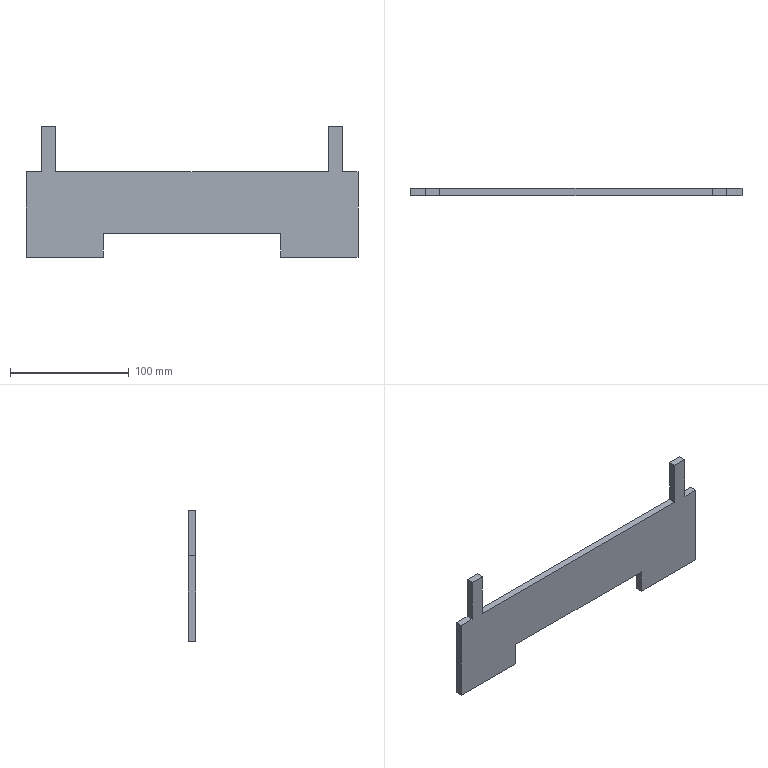Component | SolidWorks | THK-B1012LowerBaffle-1 | 1 solid | 18 faces | box 280 x 6 x 110 mm | volume 108432 mm3 | plane 18 | material Q235A
STEP:
#1=COLOUR_RGB('',0.7922,0.8196,0.9333);
#2=FILL_AREA_STYLE_COLOUR('',#1);
#3=FILL_AREA_STYLE('',(#2));
#4=SURFACE_STYLE_FILL_AREA(#3);
#5=SURFACE_SIDE_STYLE('',(#4));
#6=SURFACE_STYLE_USAGE(.BOTH.,#5);
#7=PRESENTATION_STYLE_ASSIGNMENT((#6));
#8=CARTESIAN_POINT('',(-5.,-5.354,-5.709));
#9=VERTEX_POINT('',#8);
#10=CARTESIAN_POINT('',(-4.528,-5.354,-5.709));
#11=VERTEX_POINT('',#10);
#12=CARTESIAN_POINT('',(-5.512,-5.354,-5.709));
#13=DIRECTION('',(1.,0.,0.));
#14=VECTOR('',#13,39.37);
#15=LINE('',#12,#14);
#16=EDGE_CURVE('',#9,#11,#15,.T.);
#17=ORIENTED_EDGE('',*,*,#16,.T.);
#18=CARTESIAN_POINT('',(-4.528,-5.118,-5.709));
#19=VERTEX_POINT('',#18);
#20=CARTESIAN_POINT('',(-4.528,-5.118,-5.709));
#21=DIRECTION('',(-0.,1.,0.));
#22=VECTOR('',#21,39.37);
#23=LINE('',#20,#22);
#24=EDGE_CURVE('',#11,#19,#23,.T.);
#25=ORIENTED_EDGE('',*,*,#24,.T.);
#26=CARTESIAN_POINT('',(-5.,-5.118,-5.709));
#27=VERTEX_POINT('',#26);
#28=CARTESIAN_POINT('',(-5.512,-5.118,-5.709));
#29=DIRECTION('',(1.,0.,0.));
#30=VECTOR('',#29,39.37);
#31=LINE('',#28,#30);
#32=EDGE_CURVE('',#27,#19,#31,.T.);
#33=ORIENTED_EDGE('',*,*,#32,.F.);
#34=CARTESIAN_POINT('',(-5.,-5.354,-5.709));
#35=DIRECTION('',(-0.,1.,0.));
#36=VECTOR('',#35,39.37);
#37=LINE('',#34,#36);
#38=EDGE_CURVE('',#9,#27,#37,.T.);
#39=ORIENTED_EDGE('',*,*,#38,.F.);
#40=EDGE_LOOP('',(#17,#25,#33,#39));
#41=FACE_OUTER_BOUND('',#40,.T.);
#42=CARTESIAN_POINT('',(0.,-5.118,-5.709));
#43=DIRECTION('',(0.,0.,-1.));
#44=DIRECTION('',(-1.,0.,0.));
#45=AXIS2_PLACEMENT_3D('',#42,#43,#44);
#46=PLANE('',#45);
#47=ADVANCED_FACE('',(#41),#46,.F.);
#48=CARTESIAN_POINT('',(-2.953,-5.354,-10.039));
#49=VERTEX_POINT('',#48);
#50=CARTESIAN_POINT('',(-2.953,-5.118,-10.039));
#51=VERTEX_POINT('',#50);
#52=CARTESIAN_POINT('',(-2.953,-5.118,-10.039));
#53=DIRECTION('',(-0.,1.,0.));
#54=VECTOR('',#53,39.37);
#55=LINE('',#52,#54);
#56=EDGE_CURVE('',#49,#51,#55,.T.);
#57=ORIENTED_EDGE('',*,*,#56,.F.);
#58=CARTESIAN_POINT('',(-5.512,-5.354,-10.039));
#59=VERTEX_POINT('',#58);
#60=CARTESIAN_POINT('',(-5.512,-5.354,-10.039));
#61=DIRECTION('',(1.,0.,0.));
#62=VECTOR('',#61,39.37);
#63=LINE('',#60,#62);
#64=EDGE_CURVE('',#59,#49,#63,.T.);
#65=ORIENTED_EDGE('',*,*,#64,.F.);
#66=CARTESIAN_POINT('',(-5.512,-5.118,-10.039));
#67=VERTEX_POINT('',#66);
#68=CARTESIAN_POINT('',(-5.512,-5.354,-10.039));
#69=DIRECTION('',(0.,1.,0.));
#70=VECTOR('',#69,39.37);
#71=LINE('',#68,#70);
#72=EDGE_CURVE('',#59,#67,#71,.T.);
#73=ORIENTED_EDGE('',*,*,#72,.T.);
#74=CARTESIAN_POINT('',(-5.512,-5.118,-10.039));
#75=DIRECTION('',(1.,0.,0.));
#76=VECTOR('',#75,39.37);
#77=LINE('',#74,#76);
#78=EDGE_CURVE('',#67,#51,#77,.T.);
#79=ORIENTED_EDGE('',*,*,#78,.T.);
#80=EDGE_LOOP('',(#57,#65,#73,#79));
#81=FACE_OUTER_BOUND('',#80,.T.);
#82=CARTESIAN_POINT('',(0.,-5.118,-10.039));
#83=DIRECTION('',(0.,0.,-1.));
#84=DIRECTION('',(-1.,0.,0.));
#85=AXIS2_PLACEMENT_3D('',#82,#83,#84);
#86=PLANE('',#85);
#87=ADVANCED_FACE('',(#81),#86,.T.);
#88=CARTESIAN_POINT('',(5.512,-5.354,-7.205));
#89=VERTEX_POINT('',#88);
#90=CARTESIAN_POINT('',(5.,-5.354,-7.205));
#91=VERTEX_POINT('',#90);
#92=CARTESIAN_POINT('',(5.512,-5.354,-7.205));
#93=DIRECTION('',(-1.,-0.,0.));
#94=VECTOR('',#93,39.37);
#95=LINE('',#92,#94);
#96=EDGE_CURVE('',#89,#91,#95,.T.);
#97=ORIENTED_EDGE('',*,*,#96,.T.);
#98=CARTESIAN_POINT('',(5.,-5.354,-5.709));
#99=VERTEX_POINT('',#98);
#100=CARTESIAN_POINT('',(5.,-5.354,-5.709));
#101=DIRECTION('',(0.,0.,1.));
#102=VECTOR('',#101,39.37);
#103=LINE('',#100,#102);
#104=EDGE_CURVE('',#91,#99,#103,.T.);
#105=ORIENTED_EDGE('',*,*,#104,.T.);
#106=CARTESIAN_POINT('',(4.528,-5.354,-5.709));
#107=VERTEX_POINT('',#106);
#108=CARTESIAN_POINT('',(-5.512,-5.354,-5.709));
#109=DIRECTION('',(1.,0.,0.));
#110=VECTOR('',#109,39.37);
#111=LINE('',#108,#110);
#112=EDGE_CURVE('',#107,#99,#111,.T.);
#113=ORIENTED_EDGE('',*,*,#112,.F.);
#114=CARTESIAN_POINT('',(4.528,-5.354,-7.205));
#115=VERTEX_POINT('',#114);
#116=CARTESIAN_POINT('',(4.528,-5.354,-7.205));
#117=DIRECTION('',(0.,0.,-1.));
#118=VECTOR('',#117,39.37);
#119=LINE('',#116,#118);
#120=EDGE_CURVE('',#107,#115,#119,.T.);
#121=ORIENTED_EDGE('',*,*,#120,.T.);
#122=CARTESIAN_POINT('',(-4.528,-5.354,-7.205));
#123=VERTEX_POINT('',#122);
#124=CARTESIAN_POINT('',(-4.528,-5.354,-7.205));
#125=DIRECTION('',(-1.,-0.,0.));
#126=VECTOR('',#125,39.37);
#127=LINE('',#124,#126);
#128=EDGE_CURVE('',#115,#123,#127,.T.);
#129=ORIENTED_EDGE('',*,*,#128,.T.);
#130=CARTESIAN_POINT('',(-4.528,-5.354,-7.205));
#131=DIRECTION('',(0.,0.,1.));
#132=VECTOR('',#131,39.37);
#133=LINE('',#130,#132);
#134=EDGE_CURVE('',#123,#11,#133,.T.);
#135=ORIENTED_EDGE('',*,*,#134,.T.);
#136=ORIENTED_EDGE('',*,*,#16,.F.);
#137=CARTESIAN_POINT('',(-5.,-5.354,-7.205));
#138=VERTEX_POINT('',#137);
#139=CARTESIAN_POINT('',(-5.,-5.354,-5.709));
#140=DIRECTION('',(0.,0.,-1.));
#141=VECTOR('',#140,39.37);
#142=LINE('',#139,#141);
#143=EDGE_CURVE('',#9,#138,#142,.T.);
#144=ORIENTED_EDGE('',*,*,#143,.T.);
#145=CARTESIAN_POINT('',(-5.512,-5.354,-7.205));
#146=VERTEX_POINT('',#145);
#147=CARTESIAN_POINT('',(-5.512,-5.354,-7.205));
#148=DIRECTION('',(-1.,-0.,0.));
#149=VECTOR('',#148,39.37);
#150=LINE('',#147,#149);
#151=EDGE_CURVE('',#138,#146,#150,.T.);
#152=ORIENTED_EDGE('',*,*,#151,.T.);
#153=CARTESIAN_POINT('',(-5.512,-5.354,-5.709));
#154=DIRECTION('',(0.,0.,-1.));
#155=VECTOR('',#154,39.37);
#156=LINE('',#153,#155);
#157=EDGE_CURVE('',#146,#59,#156,.T.);
#158=ORIENTED_EDGE('',*,*,#157,.T.);
#159=ORIENTED_EDGE('',*,*,#64,.T.);
#160=CARTESIAN_POINT('',(-2.953,-5.354,-9.252));
#161=VERTEX_POINT('',#160);
#162=CARTESIAN_POINT('',(-2.953,-5.354,-9.252));
#163=DIRECTION('',(0.,0.,1.));
#164=VECTOR('',#163,39.37);
#165=LINE('',#162,#164);
#166=EDGE_CURVE('',#49,#161,#165,.T.);
#167=ORIENTED_EDGE('',*,*,#166,.T.);
#168=CARTESIAN_POINT('',(2.953,-5.354,-9.252));
#169=VERTEX_POINT('',#168);
#170=CARTESIAN_POINT('',(-2.953,-5.354,-9.252));
#171=DIRECTION('',(1.,0.,0.));
#172=VECTOR('',#171,39.37);
#173=LINE('',#170,#172);
#174=EDGE_CURVE('',#161,#169,#173,.T.);
#175=ORIENTED_EDGE('',*,*,#174,.T.);
#176=CARTESIAN_POINT('',(2.953,-5.354,-10.039));
#177=VERTEX_POINT('',#176);
#178=CARTESIAN_POINT('',(2.953,-5.354,-9.252));
#179=DIRECTION('',(0.,0.,-1.));
#180=VECTOR('',#179,39.37);
#181=LINE('',#178,#180);
#182=EDGE_CURVE('',#169,#177,#181,.T.);
#183=ORIENTED_EDGE('',*,*,#182,.T.);
#184=CARTESIAN_POINT('',(5.512,-5.354,-10.039));
#185=VERTEX_POINT('',#184);
#186=CARTESIAN_POINT('',(-5.512,-5.354,-10.039));
#187=DIRECTION('',(1.,0.,0.));
#188=VECTOR('',#187,39.37);
#189=LINE('',#186,#188);
#190=EDGE_CURVE('',#177,#185,#189,.T.);
#191=ORIENTED_EDGE('',*,*,#190,.T.);
#192=CARTESIAN_POINT('',(5.512,-5.354,-5.709));
#193=DIRECTION('',(0.,0.,-1.));
#194=VECTOR('',#193,39.37);
#195=LINE('',#192,#194);
#196=EDGE_CURVE('',#89,#185,#195,.T.);
#197=ORIENTED_EDGE('',*,*,#196,.F.);
#198=EDGE_LOOP('',(#97,#105,#113,#121,#129,#135,#136,#144,#152,#158,#159,#167,#175,#183,#191,#197));
#199=FACE_OUTER_BOUND('',#198,.T.);
#200=CARTESIAN_POINT('',(-5.512,-5.354,-5.709));
#201=DIRECTION('',(-0.,1.,0.));
#202=DIRECTION('',(-1.,-0.,0.));
#203=AXIS2_PLACEMENT_3D('',#200,#201,#202);
#204=PLANE('',#203);
#205=ADVANCED_FACE('',(#199),#204,.F.);
#206=CARTESIAN_POINT('',(5.512,-5.118,-7.205));
#207=VERTEX_POINT('',#206);
#208=CARTESIAN_POINT('',(5.512,-5.354,-7.205));
#209=DIRECTION('',(-0.,1.,0.));
#210=VECTOR('',#209,39.37);
#211=LINE('',#208,#210);
#212=EDGE_CURVE('',#89,#207,#211,.T.);
#213=ORIENTED_EDGE('',*,*,#212,.F.);
#214=ORIENTED_EDGE('',*,*,#196,.T.);
#215=CARTESIAN_POINT('',(5.512,-5.118,-10.039));
#216=VERTEX_POINT('',#215);
#217=CARTESIAN_POINT('',(5.512,-5.118,-10.039));
#218=DIRECTION('',(0.,-1.,0.));
#219=VECTOR('',#218,39.37);
#220=LINE('',#217,#219);
#221=EDGE_CURVE('',#216,#185,#220,.T.);
#222=ORIENTED_EDGE('',*,*,#221,.F.);
#223=CARTESIAN_POINT('',(5.512,-5.118,-5.709));
#224=DIRECTION('',(0.,0.,-1.));
#225=VECTOR('',#224,39.37);
#226=LINE('',#223,#225);
#227=EDGE_CURVE('',#207,#216,#226,.T.);
#228=ORIENTED_EDGE('',*,*,#227,.F.);
#229=EDGE_LOOP('',(#213,#214,#222,#228));
#230=FACE_OUTER_BOUND('',#229,.T.);
#231=CARTESIAN_POINT('',(5.512,-5.118,-5.709));
#232=DIRECTION('',(1.,0.,0.));
#233=DIRECTION('',(0.,0.,-1.));
#234=AXIS2_PLACEMENT_3D('',#231,#232,#233);
#235=PLANE('',#234);
#236=ADVANCED_FACE('',(#230),#235,.T.);
#237=CARTESIAN_POINT('',(5.,-5.118,-7.205));
#238=VERTEX_POINT('',#237);
#239=CARTESIAN_POINT('',(5.,-5.118,-5.709));
#240=VERTEX_POINT('',#239);
#241=CARTESIAN_POINT('',(5.,-5.118,-5.709));
#242=DIRECTION('',(0.,0.,1.));
#243=VECTOR('',#242,39.37);
#244=LINE('',#241,#243);
#245=EDGE_CURVE('',#238,#240,#244,.T.);
#246=ORIENTED_EDGE('',*,*,#245,.F.);
#247=CARTESIAN_POINT('',(5.512,-5.118,-7.205));
#248=DIRECTION('',(-1.,-0.,0.));
#249=VECTOR('',#248,39.37);
#250=LINE('',#247,#249);
#251=EDGE_CURVE('',#207,#238,#250,.T.);
#252=ORIENTED_EDGE('',*,*,#251,.F.);
#253=ORIENTED_EDGE('',*,*,#227,.T.);
#254=CARTESIAN_POINT('',(2.953,-5.118,-10.039));
#255=VERTEX_POINT('',#254);
#256=CARTESIAN_POINT('',(-5.512,-5.118,-10.039));
#257=DIRECTION('',(1.,0.,0.));
#258=VECTOR('',#257,39.37);
#259=LINE('',#256,#258);
#260=EDGE_CURVE('',#255,#216,#259,.T.);
#261=ORIENTED_EDGE('',*,*,#260,.F.);
#262=CARTESIAN_POINT('',(2.953,-5.118,-9.252));
#263=VERTEX_POINT('',#262);
#264=CARTESIAN_POINT('',(2.953,-5.118,-9.252));
#265=DIRECTION('',(0.,0.,-1.));
#266=VECTOR('',#265,39.37);
#267=LINE('',#264,#266);
#268=EDGE_CURVE('',#263,#255,#267,.T.);
#269=ORIENTED_EDGE('',*,*,#268,.F.);
#270=CARTESIAN_POINT('',(-2.953,-5.118,-9.252));
#271=VERTEX_POINT('',#270);
#272=CARTESIAN_POINT('',(-2.953,-5.118,-9.252));
#273=DIRECTION('',(1.,0.,0.));
#274=VECTOR('',#273,39.37);
#275=LINE('',#272,#274);
#276=EDGE_CURVE('',#271,#263,#275,.T.);
#277=ORIENTED_EDGE('',*,*,#276,.F.);
#278=CARTESIAN_POINT('',(-2.953,-5.118,-9.252));
#279=DIRECTION('',(0.,0.,1.));
#280=VECTOR('',#279,39.37);
#281=LINE('',#278,#280);
#282=EDGE_CURVE('',#51,#271,#281,.T.);
#283=ORIENTED_EDGE('',*,*,#282,.F.);
#284=ORIENTED_EDGE('',*,*,#78,.F.);
#285=CARTESIAN_POINT('',(-5.512,-5.118,-7.205));
#286=VERTEX_POINT('',#285);
#287=CARTESIAN_POINT('',(-5.512,-5.118,-5.709));
#288=DIRECTION('',(0.,0.,-1.));
#289=VECTOR('',#288,39.37);
#290=LINE('',#287,#289);
#291=EDGE_CURVE('',#286,#67,#290,.T.);
#292=ORIENTED_EDGE('',*,*,#291,.F.);
#293=CARTESIAN_POINT('',(-5.,-5.118,-7.205));
#294=VERTEX_POINT('',#293);
#295=CARTESIAN_POINT('',(-5.512,-5.118,-7.205));
#296=DIRECTION('',(-1.,-0.,0.));
#297=VECTOR('',#296,39.37);
#298=LINE('',#295,#297);
#299=EDGE_CURVE('',#294,#286,#298,.T.);
#300=ORIENTED_EDGE('',*,*,#299,.F.);
#301=CARTESIAN_POINT('',(-5.,-5.118,-5.709));
#302=DIRECTION('',(0.,0.,-1.));
#303=VECTOR('',#302,39.37);
#304=LINE('',#301,#303);
#305=EDGE_CURVE('',#27,#294,#304,.T.);
#306=ORIENTED_EDGE('',*,*,#305,.F.);
#307=ORIENTED_EDGE('',*,*,#32,.T.);
#308=CARTESIAN_POINT('',(-4.528,-5.118,-7.205));
#309=VERTEX_POINT('',#308);
#310=CARTESIAN_POINT('',(-4.528,-5.118,-7.205));
#311=DIRECTION('',(0.,0.,1.));
#312=VECTOR('',#311,39.37);
#313=LINE('',#310,#312);
#314=EDGE_CURVE('',#309,#19,#313,.T.);
#315=ORIENTED_EDGE('',*,*,#314,.F.);
#316=CARTESIAN_POINT('',(4.528,-5.118,-7.205));
#317=VERTEX_POINT('',#316);
#318=CARTESIAN_POINT('',(-4.528,-5.118,-7.205));
#319=DIRECTION('',(-1.,-0.,0.));
#320=VECTOR('',#319,39.37);
#321=LINE('',#318,#320);
#322=EDGE_CURVE('',#317,#309,#321,.T.);
#323=ORIENTED_EDGE('',*,*,#322,.F.);
#324=CARTESIAN_POINT('',(4.528,-5.118,-5.709));
#325=VERTEX_POINT('',#324);
#326=CARTESIAN_POINT('',(4.528,-5.118,-7.205));
#327=DIRECTION('',(0.,0.,-1.));
#328=VECTOR('',#327,39.37);
#329=LINE('',#326,#328);
#330=EDGE_CURVE('',#325,#317,#329,.T.);
#331=ORIENTED_EDGE('',*,*,#330,.F.);
#332=CARTESIAN_POINT('',(-5.512,-5.118,-5.709));
#333=DIRECTION('',(1.,0.,0.));
#334=VECTOR('',#333,39.37);
#335=LINE('',#332,#334);
#336=EDGE_CURVE('',#325,#240,#335,.T.);
#337=ORIENTED_EDGE('',*,*,#336,.T.);
#338=EDGE_LOOP('',(#246,#252,#253,#261,#269,#277,#283,#284,#292,#300,#306,#307,#315,#323,#331,#337));
#339=FACE_OUTER_BOUND('',#338,.T.);
#340=CARTESIAN_POINT('',(-5.512,-5.118,-5.709));
#341=DIRECTION('',(-0.,1.,0.));
#342=DIRECTION('',(-1.,-0.,0.));
#343=AXIS2_PLACEMENT_3D('',#340,#341,#342);
#344=PLANE('',#343);
#345=ADVANCED_FACE('',(#339),#344,.T.);
#346=CARTESIAN_POINT('',(-5.512,-5.354,-7.205));
#347=DIRECTION('',(-0.,1.,0.));
#348=VECTOR('',#347,39.37);
#349=LINE('',#346,#348);
#350=EDGE_CURVE('',#146,#286,#349,.T.);
#351=ORIENTED_EDGE('',*,*,#350,.T.);
#352=ORIENTED_EDGE('',*,*,#291,.T.);
#353=ORIENTED_EDGE('',*,*,#72,.F.);
#354=ORIENTED_EDGE('',*,*,#157,.F.);
#355=EDGE_LOOP('',(#351,#352,#353,#354));
#356=FACE_OUTER_BOUND('',#355,.T.);
#357=CARTESIAN_POINT('',(-5.512,-5.354,-5.709));
#358=DIRECTION('',(-1.,0.,0.));
#359=DIRECTION('',(0.,0.,1.));
#360=AXIS2_PLACEMENT_3D('',#357,#358,#359);
#361=PLANE('',#360);
#362=ADVANCED_FACE('',(#356),#361,.T.);
#363=ORIENTED_EDGE('',*,*,#112,.T.);
#364=CARTESIAN_POINT('',(5.,-5.354,-5.709));
#365=DIRECTION('',(-0.,1.,0.));
#366=VECTOR('',#365,39.37);
#367=LINE('',#364,#366);
#368=EDGE_CURVE('',#99,#240,#367,.T.);
#369=ORIENTED_EDGE('',*,*,#368,.T.);
#370=ORIENTED_EDGE('',*,*,#336,.F.);
#371=CARTESIAN_POINT('',(4.528,-5.118,-5.709));
#372=DIRECTION('',(0.,-1.,0.));
#373=VECTOR('',#372,39.37);
#374=LINE('',#371,#373);
#375=EDGE_CURVE('',#325,#107,#374,.T.);
#376=ORIENTED_EDGE('',*,*,#375,.T.);
#377=EDGE_LOOP('',(#363,#369,#370,#376));
#378=FACE_OUTER_BOUND('',#377,.T.);
#379=CARTESIAN_POINT('',(0.,-5.118,-5.709));
#380=DIRECTION('',(0.,0.,-1.));
#381=DIRECTION('',(-1.,0.,0.));
#382=AXIS2_PLACEMENT_3D('',#379,#380,#381);
#383=PLANE('',#382);
#384=ADVANCED_FACE('',(#378),#383,.F.);
#385=CARTESIAN_POINT('',(2.953,-5.118,-10.039));
#386=DIRECTION('',(0.,-1.,0.));
#387=VECTOR('',#386,39.37);
#388=LINE('',#385,#387);
#389=EDGE_CURVE('',#255,#177,#388,.T.);
#390=ORIENTED_EDGE('',*,*,#389,.F.);
#391=ORIENTED_EDGE('',*,*,#260,.T.);
#392=ORIENTED_EDGE('',*,*,#221,.T.);
#393=ORIENTED_EDGE('',*,*,#190,.F.);
#394=EDGE_LOOP('',(#390,#391,#392,#393));
#395=FACE_OUTER_BOUND('',#394,.T.);
#396=CARTESIAN_POINT('',(0.,-5.118,-10.039));
#397=DIRECTION('',(0.,0.,-1.));
#398=DIRECTION('',(-1.,0.,0.));
#399=AXIS2_PLACEMENT_3D('',#396,#397,#398);
#400=PLANE('',#399);
#401=ADVANCED_FACE('',(#395),#400,.T.);
#402=ORIENTED_EDGE('',*,*,#56,.T.);
#403=ORIENTED_EDGE('',*,*,#282,.T.);
#404=CARTESIAN_POINT('',(-2.953,-5.354,-9.252));
#405=DIRECTION('',(-0.,1.,0.));
#406=VECTOR('',#405,39.37);
#407=LINE('',#404,#406);
#408=EDGE_CURVE('',#161,#271,#407,.T.);
#409=ORIENTED_EDGE('',*,*,#408,.F.);
#410=ORIENTED_EDGE('',*,*,#166,.F.);
#411=EDGE_LOOP('',(#402,#403,#409,#410));
#412=FACE_OUTER_BOUND('',#411,.T.);
#413=CARTESIAN_POINT('',(-2.953,-5.354,-9.252));
#414=DIRECTION('',(-1.,-0.,0.));
#415=DIRECTION('',(0.,-1.,0.));
#416=AXIS2_PLACEMENT_3D('',#413,#414,#415);
#417=PLANE('',#416);
#418=ADVANCED_FACE('',(#412),#417,.F.);
#419=ORIENTED_EDGE('',*,*,#389,.T.);
#420=ORIENTED_EDGE('',*,*,#182,.F.);
#421=CARTESIAN_POINT('',(2.953,-5.354,-9.252));
#422=DIRECTION('',(-0.,1.,0.));
#423=VECTOR('',#422,39.37);
#424=LINE('',#421,#423);
#425=EDGE_CURVE('',#169,#263,#424,.T.);
#426=ORIENTED_EDGE('',*,*,#425,.T.);
#427=ORIENTED_EDGE('',*,*,#268,.T.);
#428=EDGE_LOOP('',(#419,#420,#426,#427));
#429=FACE_OUTER_BOUND('',#428,.T.);
#430=CARTESIAN_POINT('',(2.953,-5.354,-9.252));
#431=DIRECTION('',(1.,0.,0.));
#432=DIRECTION('',(-0.,1.,0.));
#433=AXIS2_PLACEMENT_3D('',#430,#431,#432);
#434=PLANE('',#433);
#435=ADVANCED_FACE('',(#429),#434,.F.);
#436=ORIENTED_EDGE('',*,*,#276,.T.);
#437=ORIENTED_EDGE('',*,*,#425,.F.);
#438=ORIENTED_EDGE('',*,*,#174,.F.);
#439=ORIENTED_EDGE('',*,*,#408,.T.);
#440=EDGE_LOOP('',(#436,#437,#438,#439));
#441=FACE_OUTER_BOUND('',#440,.T.);
#442=CARTESIAN_POINT('',(-2.953,-5.354,-9.252));
#443=DIRECTION('',(0.,0.,1.));
#444=DIRECTION('',(1.,0.,0.));
#445=AXIS2_PLACEMENT_3D('',#442,#443,#444);
#446=PLANE('',#445);
#447=ADVANCED_FACE('',(#441),#446,.F.);
#448=ORIENTED_EDGE('',*,*,#299,.T.);
#449=ORIENTED_EDGE('',*,*,#350,.F.);
#450=ORIENTED_EDGE('',*,*,#151,.F.);
#451=CARTESIAN_POINT('',(-5.,-5.354,-7.205));
#452=DIRECTION('',(-0.,1.,0.));
#453=VECTOR('',#452,39.37);
#454=LINE('',#451,#453);
#455=EDGE_CURVE('',#138,#294,#454,.T.);
#456=ORIENTED_EDGE('',*,*,#455,.T.);
#457=EDGE_LOOP('',(#448,#449,#450,#456));
#458=FACE_OUTER_BOUND('',#457,.T.);
#459=CARTESIAN_POINT('',(-5.512,-5.354,-7.205));
#460=DIRECTION('',(0.,0.,-1.));
#461=DIRECTION('',(-1.,0.,0.));
#462=AXIS2_PLACEMENT_3D('',#459,#460,#461);
#463=PLANE('',#462);
#464=ADVANCED_FACE('',(#458),#463,.F.);
#465=ORIENTED_EDGE('',*,*,#305,.T.);
#466=ORIENTED_EDGE('',*,*,#455,.F.);
#467=ORIENTED_EDGE('',*,*,#143,.F.);
#468=ORIENTED_EDGE('',*,*,#38,.T.);
#469=EDGE_LOOP('',(#465,#466,#467,#468));
#470=FACE_OUTER_BOUND('',#469,.T.);
#471=CARTESIAN_POINT('',(-5.,-5.354,-5.709));
#472=DIRECTION('',(1.,0.,0.));
#473=DIRECTION('',(-0.,1.,0.));
#474=AXIS2_PLACEMENT_3D('',#471,#472,#473);
#475=PLANE('',#474);
#476=ADVANCED_FACE('',(#470),#475,.F.);
#477=ORIENTED_EDGE('',*,*,#134,.F.);
#478=CARTESIAN_POINT('',(-4.528,-5.354,-7.205));
#479=DIRECTION('',(-0.,1.,0.));
#480=VECTOR('',#479,39.37);
#481=LINE('',#478,#480);
#482=EDGE_CURVE('',#123,#309,#481,.T.);
#483=ORIENTED_EDGE('',*,*,#482,.T.);
#484=ORIENTED_EDGE('',*,*,#314,.T.);
#485=ORIENTED_EDGE('',*,*,#24,.F.);
#486=EDGE_LOOP('',(#477,#483,#484,#485));
#487=FACE_OUTER_BOUND('',#486,.T.);
#488=CARTESIAN_POINT('',(-4.528,-5.354,-7.205));
#489=DIRECTION('',(-1.,-0.,0.));
#490=DIRECTION('',(0.,0.,1.));
#491=AXIS2_PLACEMENT_3D('',#488,#489,#490);
#492=PLANE('',#491);
#493=ADVANCED_FACE('',(#487),#492,.F.);
#494=ORIENTED_EDGE('',*,*,#330,.T.);
#495=CARTESIAN_POINT('',(4.528,-5.354,-7.205));
#496=DIRECTION('',(-0.,1.,0.));
#497=VECTOR('',#496,39.37);
#498=LINE('',#495,#497);
#499=EDGE_CURVE('',#115,#317,#498,.T.);
#500=ORIENTED_EDGE('',*,*,#499,.F.);
#501=ORIENTED_EDGE('',*,*,#120,.F.);
#502=ORIENTED_EDGE('',*,*,#375,.F.);
#503=EDGE_LOOP('',(#494,#500,#501,#502));
#504=FACE_OUTER_BOUND('',#503,.T.);
#505=CARTESIAN_POINT('',(4.528,-5.354,-7.205));
#506=DIRECTION('',(1.,0.,0.));
#507=DIRECTION('',(0.,0.,-1.));
#508=AXIS2_PLACEMENT_3D('',#505,#506,#507);
#509=PLANE('',#508);
#510=ADVANCED_FACE('',(#504),#509,.F.);
#511=ORIENTED_EDGE('',*,*,#322,.T.);
#512=ORIENTED_EDGE('',*,*,#482,.F.);
#513=ORIENTED_EDGE('',*,*,#128,.F.);
#514=ORIENTED_EDGE('',*,*,#499,.T.);
#515=EDGE_LOOP('',(#511,#512,#513,#514));
#516=FACE_OUTER_BOUND('',#515,.T.);
#517=CARTESIAN_POINT('',(-4.528,-5.354,-7.205));
#518=DIRECTION('',(0.,0.,-1.));
#519=DIRECTION('',(-1.,0.,0.));
#520=AXIS2_PLACEMENT_3D('',#517,#518,#519);
#521=PLANE('',#520);
#522=ADVANCED_FACE('',(#516),#521,.F.);
#523=ORIENTED_EDGE('',*,*,#245,.T.);
#524=ORIENTED_EDGE('',*,*,#368,.F.);
#525=ORIENTED_EDGE('',*,*,#104,.F.);
#526=CARTESIAN_POINT('',(5.,-5.354,-7.205));
#527=DIRECTION('',(-0.,1.,0.));
#528=VECTOR('',#527,39.37);
#529=LINE('',#526,#528);
#530=EDGE_CURVE('',#91,#238,#529,.T.);
#531=ORIENTED_EDGE('',*,*,#530,.T.);
#532=EDGE_LOOP('',(#523,#524,#525,#531));
#533=FACE_OUTER_BOUND('',#532,.T.);
#534=CARTESIAN_POINT('',(5.,-5.354,-5.709));
#535=DIRECTION('',(-1.,-0.,0.));
#536=DIRECTION('',(0.,-1.,0.));
#537=AXIS2_PLACEMENT_3D('',#534,#535,#536);
#538=PLANE('',#537);
#539=ADVANCED_FACE('',(#533),#538,.F.);
#540=ORIENTED_EDGE('',*,*,#251,.T.);
#541=ORIENTED_EDGE('',*,*,#530,.F.);
#542=ORIENTED_EDGE('',*,*,#96,.F.);
#543=ORIENTED_EDGE('',*,*,#212,.T.);
#544=EDGE_LOOP('',(#540,#541,#542,#543));
#545=FACE_OUTER_BOUND('',#544,.T.);
#546=CARTESIAN_POINT('',(5.512,-5.354,-7.205));
#547=DIRECTION('',(0.,0.,-1.));
#548=DIRECTION('',(-1.,0.,0.));
#549=AXIS2_PLACEMENT_3D('',#546,#547,#548);
#550=PLANE('',#549);
#551=ADVANCED_FACE('',(#545),#550,.F.);
#552=CLOSED_SHELL('',(#47,#87,#205,#236,#345,#362,#384,#401,#418,#435,#447,#464,#476,#493,#510,#522,#539,#551));
#553=MANIFOLD_SOLID_BREP('',#552);
#554=STYLED_ITEM('',(#7),#553);
#555=(LENGTH_UNIT()NAMED_UNIT(*)SI_UNIT($,.METRE.));
#556=LENGTH_MEASURE_WITH_UNIT(LENGTH_MEASURE(0.0254),#555);
#557=DIMENSIONAL_EXPONENTS(1.,0.,0.,0.,0.,0.,0.);
#558=(CONVERSION_BASED_UNIT('',#556)LENGTH_UNIT()NAMED_UNIT(#557));
#559=UNCERTAINTY_MEASURE_WITH_UNIT(LENGTH_MEASURE(0.00001),#558,'','');
#560=(NAMED_UNIT(*)PLANE_ANGLE_UNIT()SI_UNIT($,.RADIAN.));
#561=(NAMED_UNIT(*)SI_UNIT($,.STERADIAN.)SOLID_ANGLE_UNIT());
#562=(GEOMETRIC_REPRESENTATION_CONTEXT(3)GLOBAL_UNCERTAINTY_ASSIGNED_CONTEXT((#559))GLOBAL_UNIT_ASSIGNED_CONTEXT((#558,#560,#561))REPRESENTATION_CONTEXT('',''));
#563=MECHANICAL_DESIGN_GEOMETRIC_PRESENTATION_REPRESENTATION('',(#554),#562);
#564=CARTESIAN_POINT('',(0.,0.,0.));
#565=DIRECTION('',(0.,0.,1.));
#566=DIRECTION('',(1.,0.,0.));
#567=AXIS2_PLACEMENT_3D('',#564,#565,#566);
#568=(LENGTH_UNIT()NAMED_UNIT(*)SI_UNIT($,.METRE.));
#569=LENGTH_MEASURE_WITH_UNIT(LENGTH_MEASURE(0.0254),#568);
#570=DIMENSIONAL_EXPONENTS(1.,0.,0.,0.,0.,0.,0.);
#571=(CONVERSION_BASED_UNIT('',#569)LENGTH_UNIT()NAMED_UNIT(#570));
#572=UNCERTAINTY_MEASURE_WITH_UNIT(LENGTH_MEASURE(0.00001),#571,'','');
#573=(NAMED_UNIT(*)PLANE_ANGLE_UNIT()SI_UNIT($,.RADIAN.));
#574=(NAMED_UNIT(*)SI_UNIT($,.STERADIAN.)SOLID_ANGLE_UNIT());
#575=(GEOMETRIC_REPRESENTATION_CONTEXT(3)GLOBAL_UNCERTAINTY_ASSIGNED_CONTEXT((#572))GLOBAL_UNIT_ASSIGNED_CONTEXT((#571,#573,#574))REPRESENTATION_CONTEXT('',''));
#576=ADVANCED_BREP_SHAPE_REPRESENTATION('',(#553,#567),#575);
#577=PRESENTATION_LAYER_ASSIGNMENT('','',(#554));